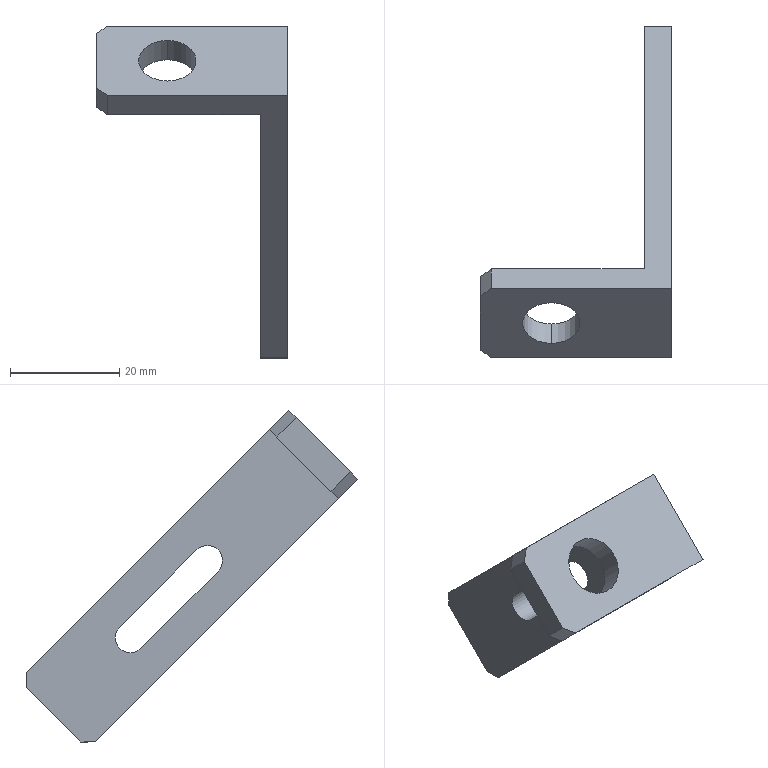Component | SolidWorks | ZL-10-06L-shapedBracket-1 | 1 solid | 19 faces | box 35 x 60.81 x 60.81 mm | volume 7858 mm3 | plane 14 | cylinder 5 | commonest cylinder face diameters 5.5 x3 10.5 x2
build123d program:
from build123d import *

# Parameters (mm, degrees)
EXTRUDE1_DEPTH     = 9
CUT_EXTRUDE1_DEPTH = 79.778
SKETCH3_R          = 5.25
CUT_EXTRUDE2_DEPTH = 79.778
CHAMFER1_SIZE      = 2


with BuildPart() as part:
    # Sketch1 → Extrude1 (new, symmetric)
    with BuildSketch(Plane.XY):
        Polygon((0, 0), (35, 0), (35, 5), (5, 5), (5, 70), (0, 70), align=None)
    extrude(amount=EXTRUDE1_DEPTH, both=True)

    # Sketch2 → Cut-Extrude1 (cut, through all)
    with BuildSketch(Plane.ZY):
        with BuildLine():
            Line((-2.75, 50), (-2.75, 30))
            ThreePointArc((-2.75, 30), (0, 27.25), (2.75, 30))
            Line((2.75, 30), (2.75, 50))
            ThreePointArc((2.75, 50), (0, 52.75), (-2.75, 50))
        make_face()
    extrude(amount=-CUT_EXTRUDE1_DEPTH, mode=Mode.SUBTRACT)

    # Sketch3 → Cut-Extrude2 (cut, through all)
    with BuildSketch(Plane.XZ):
        with Locations(Location((22, 0, 0), (0, 0, 270))):
            Circle(SKETCH3_R)
    extrude(amount=-CUT_EXTRUDE2_DEPTH, mode=Mode.SUBTRACT)

    # Chamfer1
    chamfer1_edges = [part.edges().sort_by_distance(p)[0] for p in [
        (35, 2.5, 9),
        (2.5, 70, 9),
        (2.5, 70, -9),
        (35, 2.5, -9),
    ]]
    chamfer(chamfer1_edges, length=CHAMFER1_SIZE)


solid = part.part

# Placed as in the assembly
solid = solid.moved(Location((66.323, 16.651, 28.684), (135, 0, -180)))